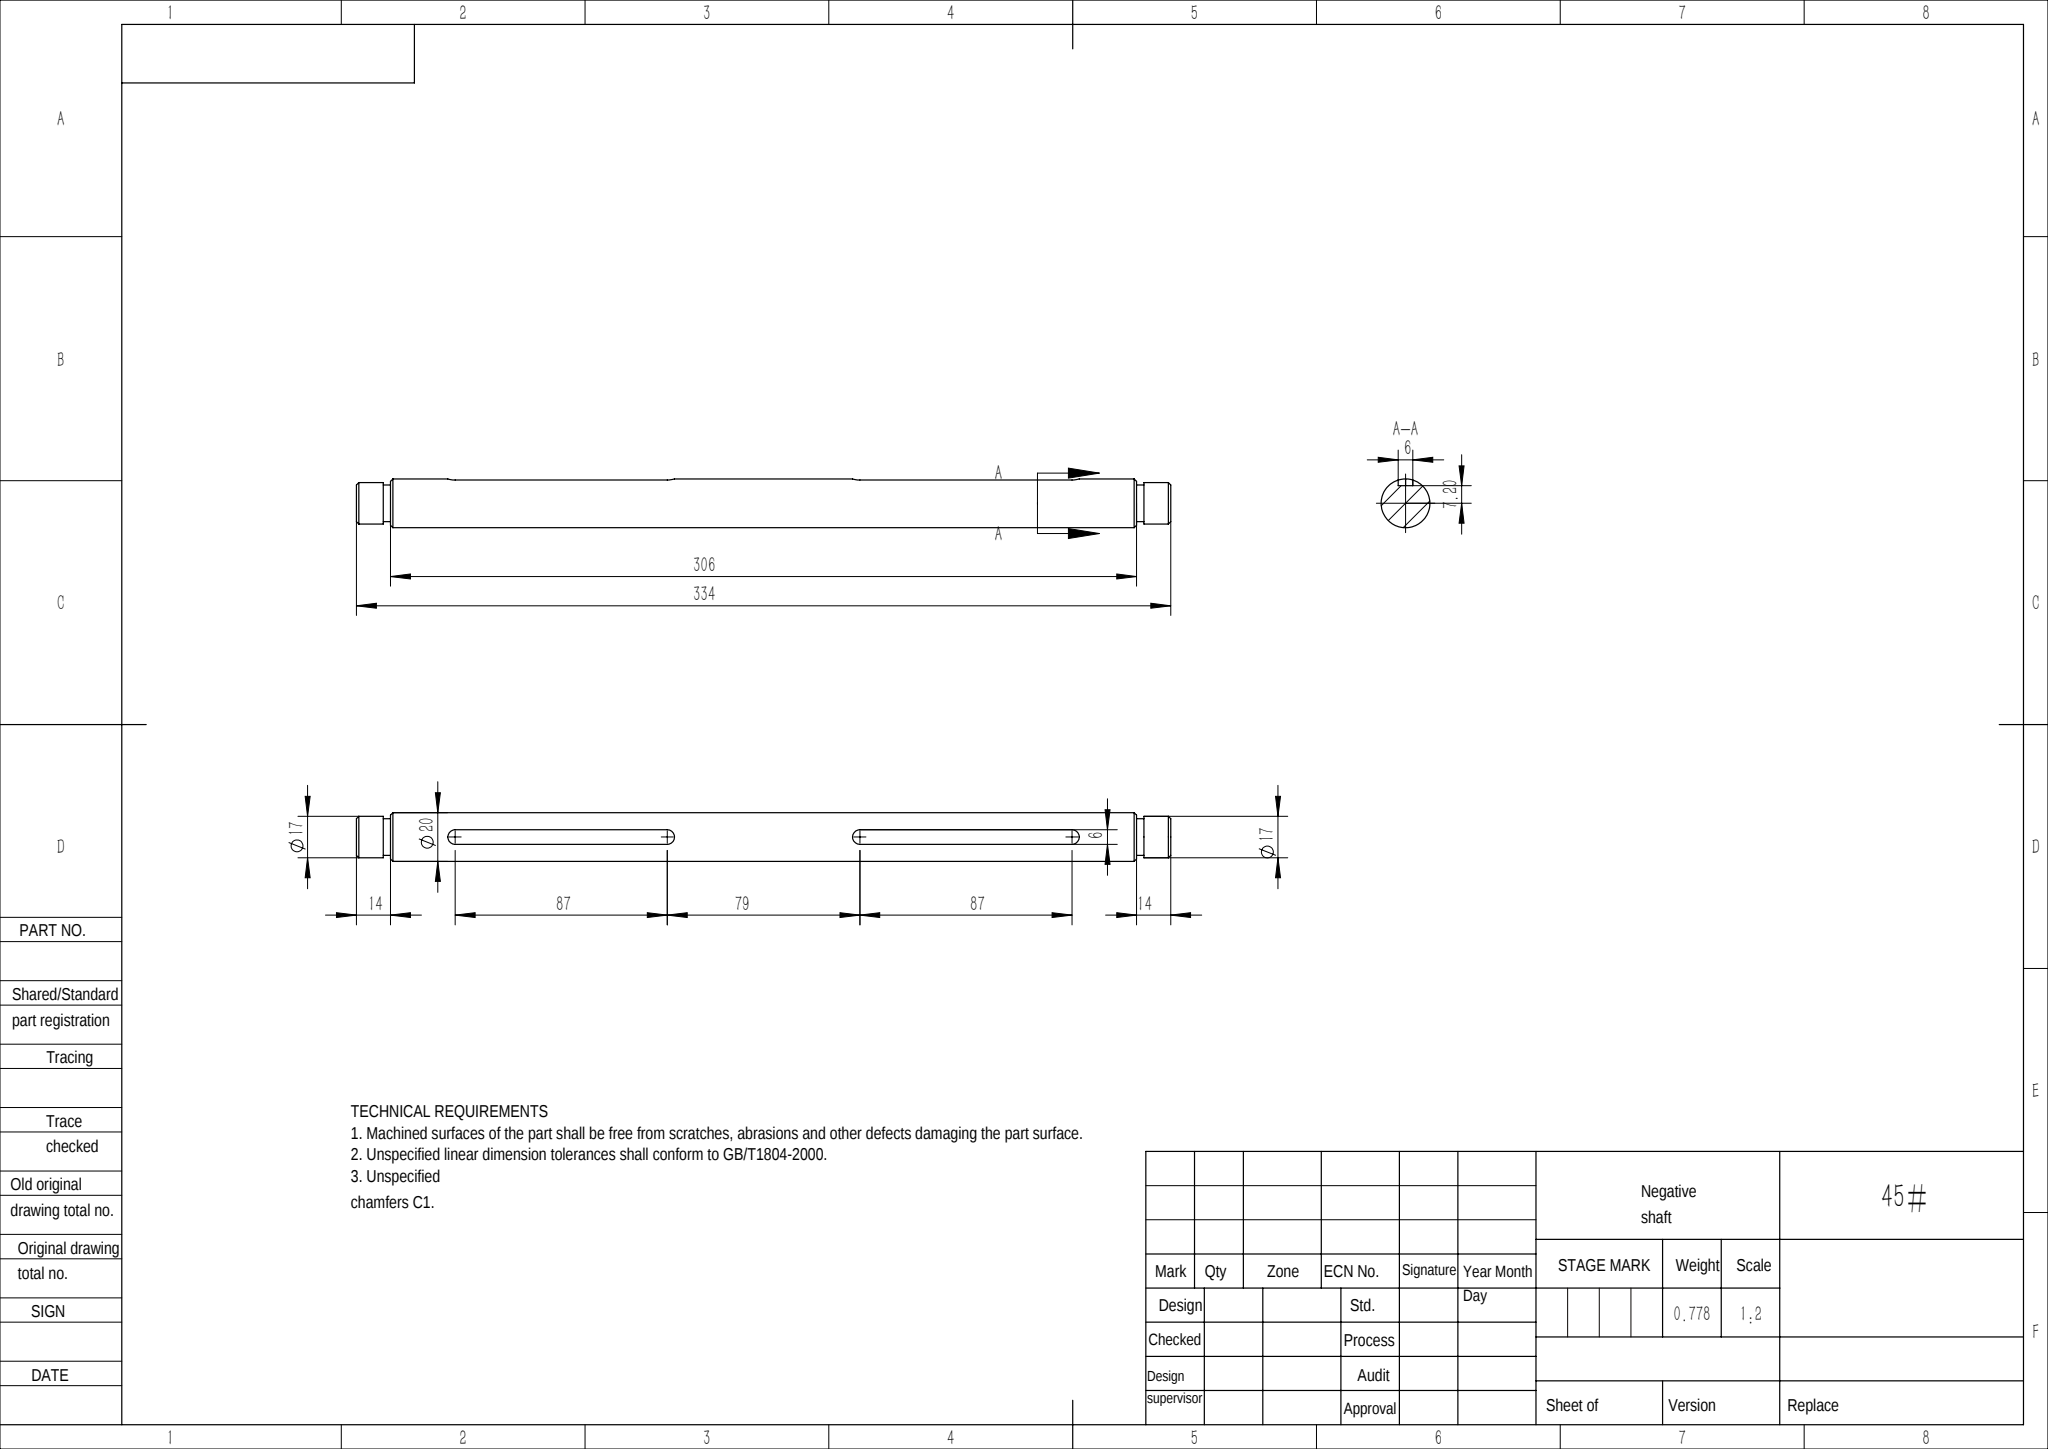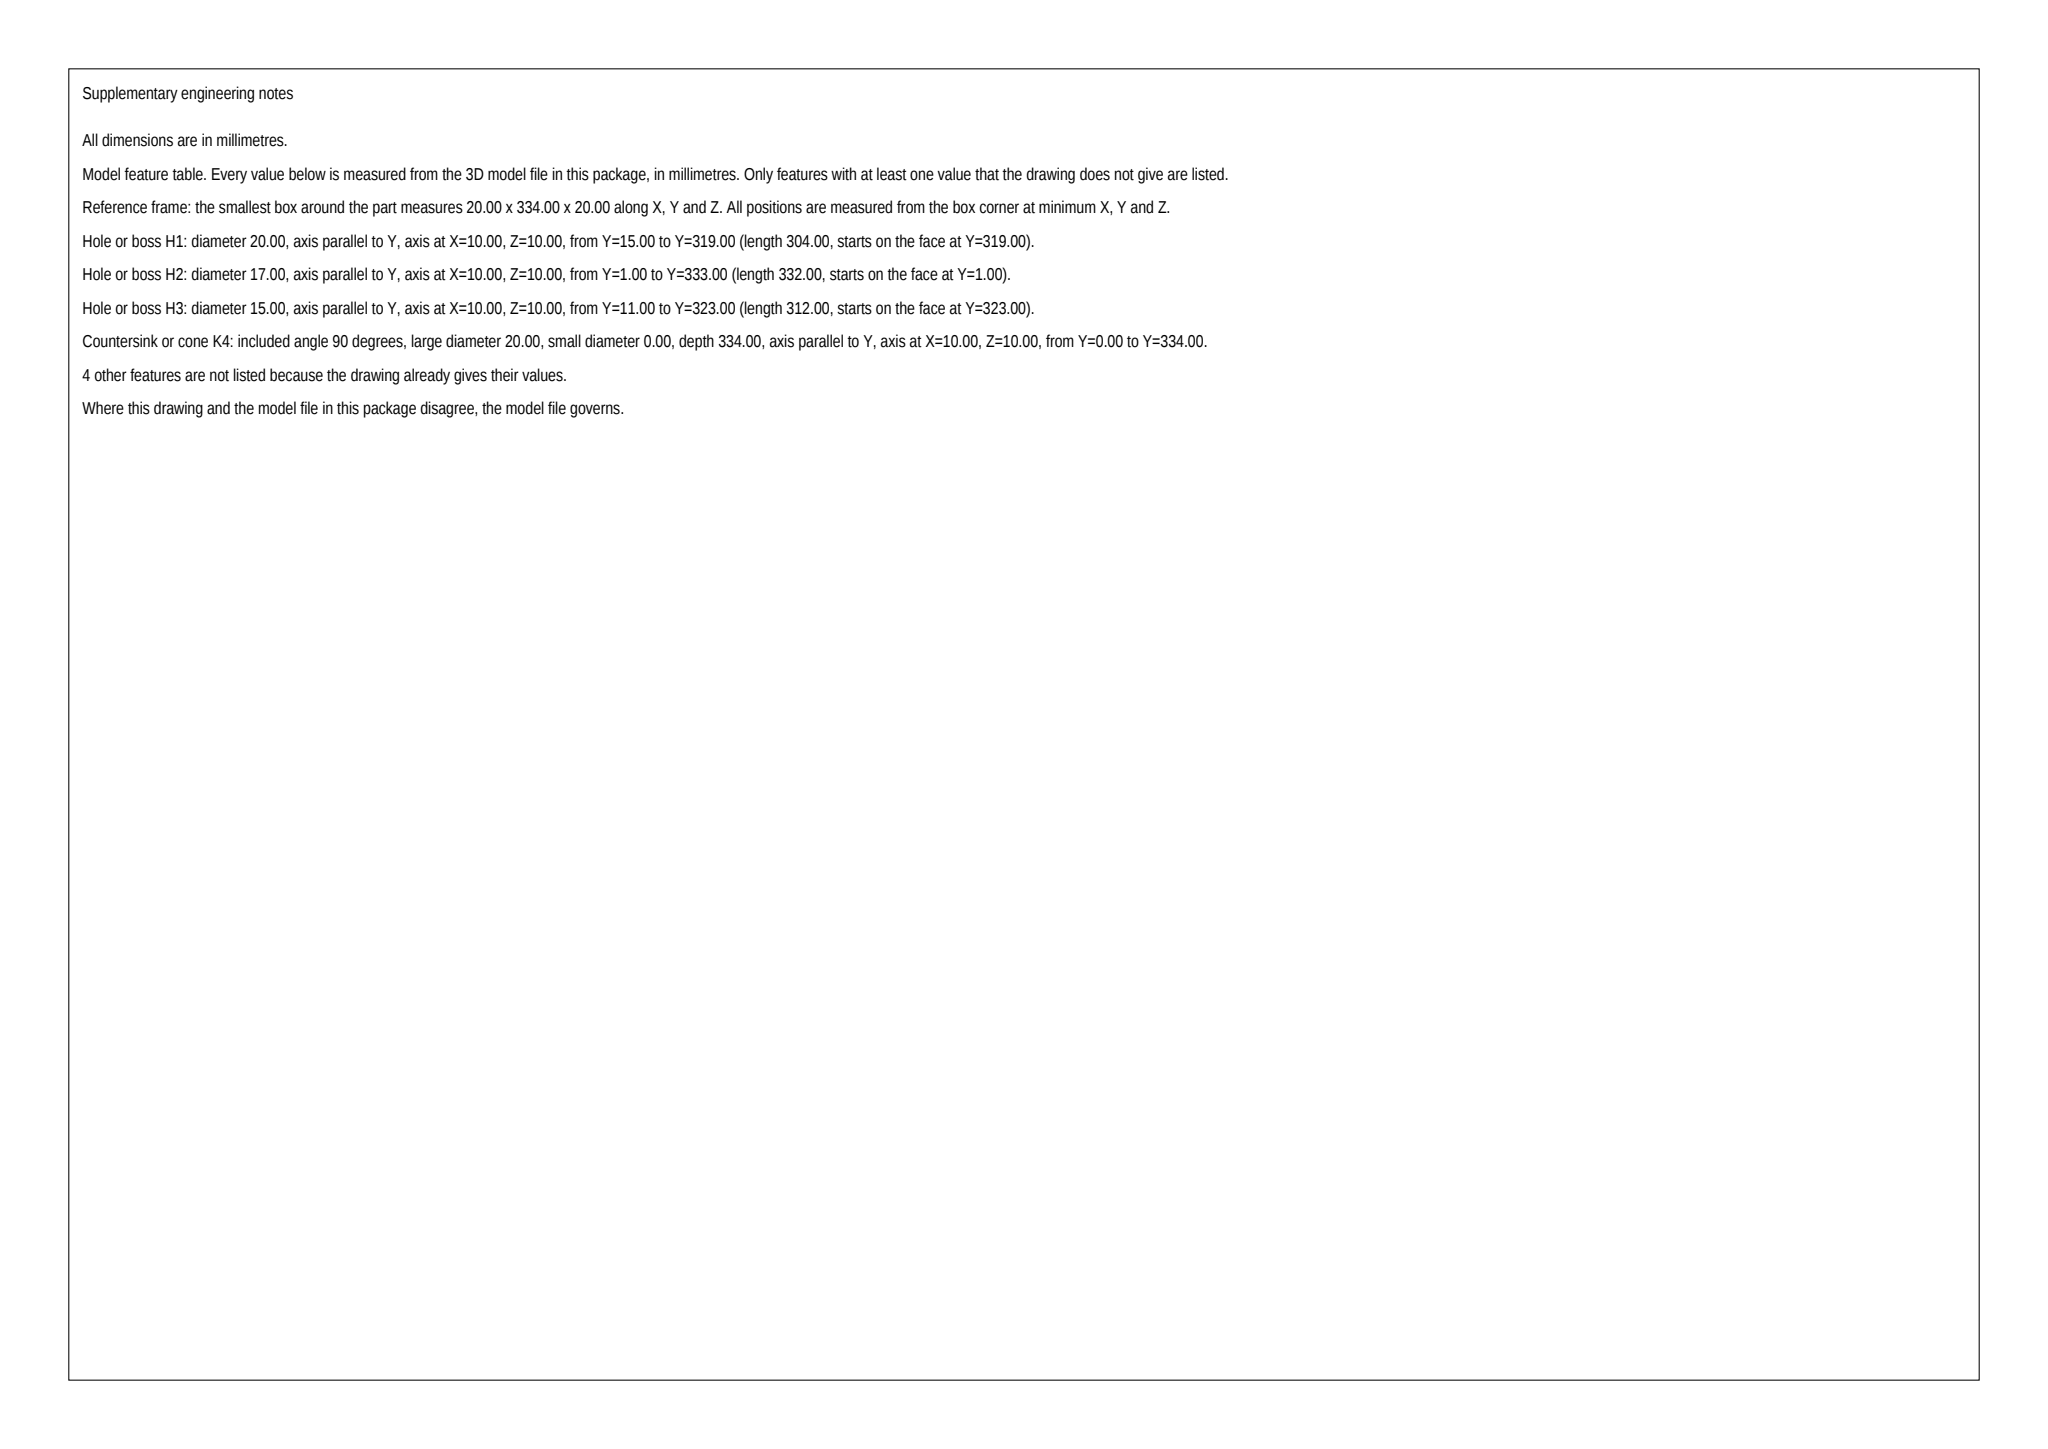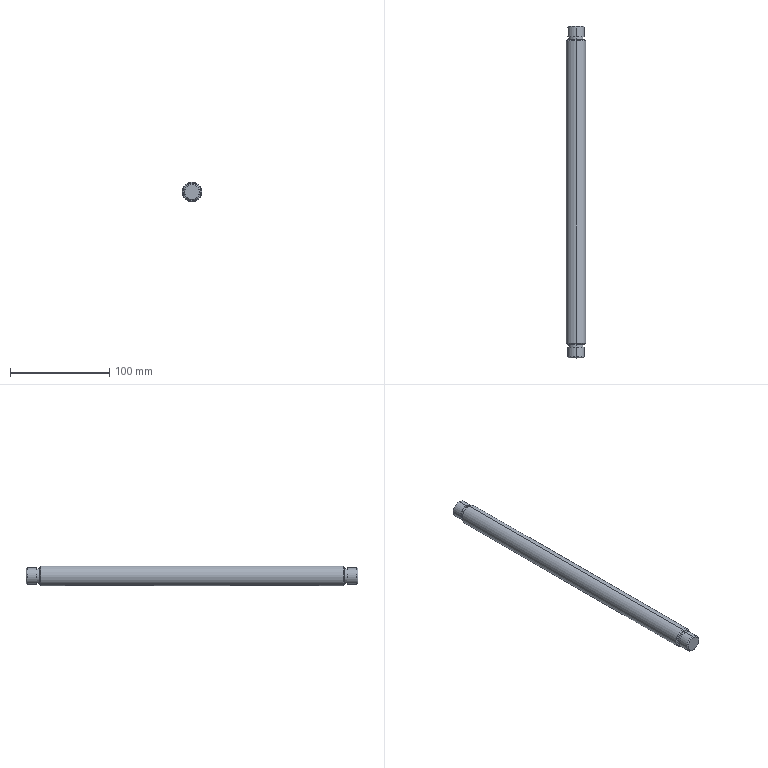Part | SolidWorks | mm | material 45# | 1 solid | 38 faces | box 20 x 334 x 20 mm | volume 99158 mm3 | cylinder 18 | plane 12 | cone 8 | commonest cylinder face diameters 6 x8 17 x4 15 x4 20 x2